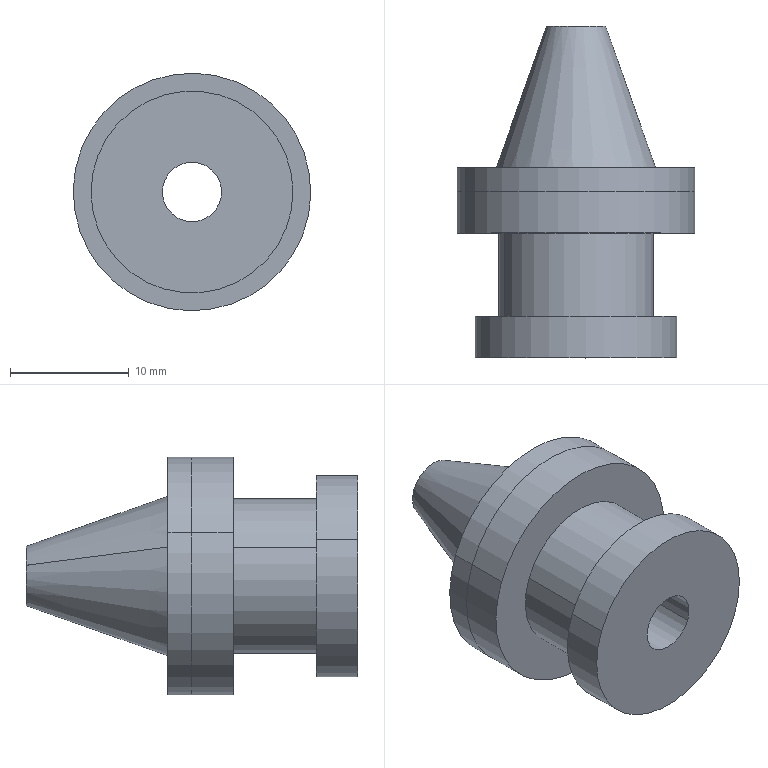Component | SolidWorks | CylinderEndCap-1 | 2 solids | 20 faces | box 20 x 27.94 x 20 mm | volume 3757 mm3 | cylinder 10 | plane 6 | cone 4 | commonest cylinder face diameters 20 x4 5 x2 17 x2 13 x2
build123d program:
from build123d import *

# Parameters (mm, degrees)
SKETCH2_R          = 2.5
CUT_EXTRUDE1_DEPTH = 38.749


with BuildPart() as part:
    # Sketch1 → Revolve1 (revolve)
    with BuildSketch(Plane.XY):
        Polygon((0, 0), (21, 7.436), (21, 10), (24.5, 10), (24.5, 6.5), (31.5, 6.5), (31.5, 8.5), (35, 8.5), (35, 0), align=None)
    revolve(axis=Axis((35, 0, 0), (-1, 0, 0)))

    # Sketch2 → Cut-Extrude1 (cut, through all)
    with BuildSketch(Plane(origin=(35, 0, 0), x_dir=(0, 0, -1), z_dir=(1, 0, 0))):
        with Locations(Location((0, 0, 0), (0, 0, 90))):
            Circle(SKETCH2_R)
    extrude(amount=-CUT_EXTRUDE1_DEPTH, mode=Mode.SUBTRACT)


with BuildPart() as body_2:
    # Sketch3 → Revolve2 (revolve)
    with BuildSketch(Plane.XY):
        Polygon((21, 10), (19, 10), (19, 6.728), (21, 7.436), align=None)
    revolve(axis=Axis((21, 0, 0), (1, 0, 0)))


solid = Compound([part.part, body_2.part])

# Placed as in the assembly
solid = solid.moved(Location((-25, -95, 0), (0, 0, -90)))
STEP:
#1=COLOUR_RGB('',0.7922,0.8196,0.9333);
#2=FILL_AREA_STYLE_COLOUR('',#1);
#3=FILL_AREA_STYLE('',(#2));
#4=SURFACE_STYLE_FILL_AREA(#3);
#5=SURFACE_SIDE_STYLE('',(#4));
#6=SURFACE_STYLE_USAGE(.BOTH.,#5);
#7=PRESENTATION_STYLE_ASSIGNMENT((#6));
#8=CARTESIAN_POINT('',(-0.8926,-4.018,-0.03578));
#9=VERTEX_POINT('',#8);
#10=CARTESIAN_POINT('',(-1.076,-4.018,0.03578));
#11=VERTEX_POINT('',#10);
#12=CARTESIAN_POINT('',(-0.9843,-4.018,0.));
#13=DIRECTION('',(-0.,1.,0.));
#14=DIRECTION('',(0.9316,0.,-0.3635));
#15=AXIS2_PLACEMENT_3D('',#12,#13,#14);
#16=CIRCLE('',#15,0.09843);
#17=EDGE_CURVE('',#9,#11,#16,.T.);
#18=ORIENTED_EDGE('',*,*,#17,.T.);
#19=CARTESIAN_POINT('',(-1.076,-5.118,0.03578));
#20=VERTEX_POINT('',#19);
#21=CARTESIAN_POINT('',(-1.076,-3.74,0.03578));
#22=DIRECTION('',(0.,-1.,0.));
#23=VECTOR('',#22,39.37);
#24=LINE('',#21,#23);
#25=EDGE_CURVE('',#11,#20,#24,.T.);
#26=ORIENTED_EDGE('',*,*,#25,.T.);
#27=CARTESIAN_POINT('',(-0.8926,-5.118,-0.03578));
#28=VERTEX_POINT('',#27);
#29=CARTESIAN_POINT('',(-0.9843,-5.118,0.));
#30=DIRECTION('',(0.,-1.,0.));
#31=DIRECTION('',(0.9316,0.,-0.3635));
#32=AXIS2_PLACEMENT_3D('',#29,#30,#31);
#33=CIRCLE('',#32,0.09843);
#34=EDGE_CURVE('',#20,#28,#33,.T.);
#35=ORIENTED_EDGE('',*,*,#34,.T.);
#36=CARTESIAN_POINT('',(-0.8926,-3.74,-0.03578));
#37=DIRECTION('',(0.,-1.,0.));
#38=VECTOR('',#37,39.37);
#39=LINE('',#36,#38);
#40=EDGE_CURVE('',#9,#28,#39,.T.);
#41=ORIENTED_EDGE('',*,*,#40,.F.);
#42=EDGE_LOOP('',(#18,#26,#35,#41));
#43=FACE_OUTER_BOUND('',#42,.T.);
#44=CARTESIAN_POINT('',(-0.9843,-3.74,0.));
#45=DIRECTION('',(0.,-1.,0.));
#46=DIRECTION('',(0.9316,0.,-0.3635));
#47=AXIS2_PLACEMENT_3D('',#44,#45,#46);
#48=CYLINDRICAL_SURFACE('',#47,0.09843);
#49=ADVANCED_FACE('',(#43),#48,.F.);
#50=CARTESIAN_POINT('',(-0.6725,-4.98,-0.1216));
#51=VERTEX_POINT('',#50);
#52=CARTESIAN_POINT('',(-1.296,-4.98,0.1216));
#53=VERTEX_POINT('',#52);
#54=CARTESIAN_POINT('',(-0.9843,-4.98,0.));
#55=DIRECTION('',(0.,-1.,-0.));
#56=DIRECTION('',(0.9316,0.,-0.3635));
#57=AXIS2_PLACEMENT_3D('',#54,#55,#56);
#58=CIRCLE('',#57,0.3346);
#59=EDGE_CURVE('',#51,#53,#58,.T.);
#60=ORIENTED_EDGE('',*,*,#59,.T.);
#61=CARTESIAN_POINT('',(-1.296,-5.118,0.1216));
#62=VERTEX_POINT('',#61);
#63=CARTESIAN_POINT('',(-1.296,-5.118,0.1216));
#64=DIRECTION('',(0.,-1.,-0.));
#65=VECTOR('',#64,39.37);
#66=LINE('',#63,#65);
#67=EDGE_CURVE('',#53,#62,#66,.T.);
#68=ORIENTED_EDGE('',*,*,#67,.T.);
#69=CARTESIAN_POINT('',(-0.6725,-5.118,-0.1216));
#70=VERTEX_POINT('',#69);
#71=CARTESIAN_POINT('',(-0.9843,-5.118,0.));
#72=DIRECTION('',(0.,-1.,-0.));
#73=DIRECTION('',(0.9316,0.,-0.3635));
#74=AXIS2_PLACEMENT_3D('',#71,#72,#73);
#75=CIRCLE('',#74,0.3346);
#76=EDGE_CURVE('',#70,#62,#75,.T.);
#77=ORIENTED_EDGE('',*,*,#76,.F.);
#78=CARTESIAN_POINT('',(-0.6725,-5.118,-0.1216));
#79=DIRECTION('',(0.,-1.,-0.));
#80=VECTOR('',#79,39.37);
#81=LINE('',#78,#80);
#82=EDGE_CURVE('',#51,#70,#81,.T.);
#83=ORIENTED_EDGE('',*,*,#82,.F.);
#84=EDGE_LOOP('',(#60,#68,#77,#83));
#85=FACE_OUTER_BOUND('',#84,.T.);
#86=CARTESIAN_POINT('',(-0.9843,-5.118,0.));
#87=DIRECTION('',(0.,-1.,-0.));
#88=DIRECTION('',(0.9316,0.,-0.3635));
#89=AXIS2_PLACEMENT_3D('',#86,#87,#88);
#90=CYLINDRICAL_SURFACE('',#89,0.3346);
#91=ADVANCED_FACE('',(#85),#90,.T.);
#92=CARTESIAN_POINT('',(-0.7459,-4.705,-0.09302));
#93=VERTEX_POINT('',#92);
#94=CARTESIAN_POINT('',(-1.223,-4.705,0.09302));
#95=VERTEX_POINT('',#94);
#96=CARTESIAN_POINT('',(-0.9843,-4.705,0.));
#97=DIRECTION('',(0.,-1.,-0.));
#98=DIRECTION('',(0.9316,0.,-0.3635));
#99=AXIS2_PLACEMENT_3D('',#96,#97,#98);
#100=CIRCLE('',#99,0.2559);
#101=EDGE_CURVE('',#93,#95,#100,.T.);
#102=ORIENTED_EDGE('',*,*,#101,.T.);
#103=CARTESIAN_POINT('',(-1.223,-4.98,0.09302));
#104=VERTEX_POINT('',#103);
#105=CARTESIAN_POINT('',(-1.223,-5.118,0.09302));
#106=DIRECTION('',(0.,-1.,-0.));
#107=VECTOR('',#106,39.37);
#108=LINE('',#105,#107);
#109=EDGE_CURVE('',#95,#104,#108,.T.);
#110=ORIENTED_EDGE('',*,*,#109,.T.);
#111=CARTESIAN_POINT('',(-0.7459,-4.98,-0.09302));
#112=VERTEX_POINT('',#111);
#113=CARTESIAN_POINT('',(-0.9843,-4.98,0.));
#114=DIRECTION('',(0.,-1.,-0.));
#115=DIRECTION('',(0.9316,0.,-0.3635));
#116=AXIS2_PLACEMENT_3D('',#113,#114,#115);
#117=CIRCLE('',#116,0.2559);
#118=EDGE_CURVE('',#112,#104,#117,.T.);
#119=ORIENTED_EDGE('',*,*,#118,.F.);
#120=CARTESIAN_POINT('',(-0.7459,-5.118,-0.09302));
#121=DIRECTION('',(0.,-1.,-0.));
#122=VECTOR('',#121,39.37);
#123=LINE('',#120,#122);
#124=EDGE_CURVE('',#93,#112,#123,.T.);
#125=ORIENTED_EDGE('',*,*,#124,.F.);
#126=EDGE_LOOP('',(#102,#110,#119,#125));
#127=FACE_OUTER_BOUND('',#126,.T.);
#128=CARTESIAN_POINT('',(-0.9843,-5.118,0.));
#129=DIRECTION('',(0.,-1.,-0.));
#130=DIRECTION('',(0.9316,0.,-0.3635));
#131=AXIS2_PLACEMENT_3D('',#128,#129,#130);
#132=CYLINDRICAL_SURFACE('',#131,0.2559);
#133=ADVANCED_FACE('',(#127),#132,.T.);
#134=CARTESIAN_POINT('',(-0.6175,-4.567,-0.1431));
#135=VERTEX_POINT('',#134);
#136=CARTESIAN_POINT('',(-1.351,-4.567,0.1431));
#137=VERTEX_POINT('',#136);
#138=CARTESIAN_POINT('',(-0.9843,-4.567,0.));
#139=DIRECTION('',(0.,-1.,-0.));
#140=DIRECTION('',(0.9316,0.,-0.3635));
#141=AXIS2_PLACEMENT_3D('',#138,#139,#140);
#142=CIRCLE('',#141,0.3937);
#143=EDGE_CURVE('',#135,#137,#142,.T.);
#144=ORIENTED_EDGE('',*,*,#143,.T.);
#145=CARTESIAN_POINT('',(-1.351,-4.705,0.1431));
#146=VERTEX_POINT('',#145);
#147=CARTESIAN_POINT('',(-1.351,-5.118,0.1431));
#148=DIRECTION('',(0.,-1.,-0.));
#149=VECTOR('',#148,39.37);
#150=LINE('',#147,#149);
#151=EDGE_CURVE('',#137,#146,#150,.T.);
#152=ORIENTED_EDGE('',*,*,#151,.T.);
#153=CARTESIAN_POINT('',(-0.6175,-4.705,-0.1431));
#154=VERTEX_POINT('',#153);
#155=CARTESIAN_POINT('',(-0.9843,-4.705,0.));
#156=DIRECTION('',(0.,-1.,-0.));
#157=DIRECTION('',(0.9316,0.,-0.3635));
#158=AXIS2_PLACEMENT_3D('',#155,#156,#157);
#159=CIRCLE('',#158,0.3937);
#160=EDGE_CURVE('',#154,#146,#159,.T.);
#161=ORIENTED_EDGE('',*,*,#160,.F.);
#162=CARTESIAN_POINT('',(-0.6175,-5.118,-0.1431));
#163=DIRECTION('',(0.,-1.,-0.));
#164=VECTOR('',#163,39.37);
#165=LINE('',#162,#164);
#166=EDGE_CURVE('',#135,#154,#165,.T.);
#167=ORIENTED_EDGE('',*,*,#166,.F.);
#168=EDGE_LOOP('',(#144,#152,#161,#167));
#169=FACE_OUTER_BOUND('',#168,.T.);
#170=CARTESIAN_POINT('',(-0.9843,-5.118,0.));
#171=DIRECTION('',(0.,-1.,-0.));
#172=DIRECTION('',(0.9316,0.,-0.3635));
#173=AXIS2_PLACEMENT_3D('',#170,#171,#172);
#174=CYLINDRICAL_SURFACE('',#173,0.3937);
#175=ADVANCED_FACE('',(#169),#174,.T.);
#176=CARTESIAN_POINT('',(-0.9843,-4.018,0.));
#177=DIRECTION('',(-0.,1.,0.));
#178=DIRECTION('',(0.9316,0.,-0.3635));
#179=AXIS2_PLACEMENT_3D('',#176,#177,#178);
#180=CIRCLE('',#179,0.09843);
#181=EDGE_CURVE('',#11,#9,#180,.T.);
#182=ORIENTED_EDGE('',*,*,#181,.F.);
#183=CARTESIAN_POINT('',(-1.257,-4.567,0.1064));
#184=VERTEX_POINT('',#183);
#185=CARTESIAN_POINT('',(-1.257,-4.567,0.1064));
#186=DIRECTION('',(-0.311,-0.9426,0.1213));
#187=VECTOR('',#186,39.37);
#188=LINE('',#185,#187);
#189=EDGE_CURVE('',#11,#184,#188,.T.);
#190=ORIENTED_EDGE('',*,*,#189,.T.);
#191=CARTESIAN_POINT('',(-0.7115,-4.567,-0.1064));
#192=VERTEX_POINT('',#191);
#193=CARTESIAN_POINT('',(-0.9843,-4.567,0.));
#194=DIRECTION('',(0.,-1.,-0.));
#195=DIRECTION('',(0.9316,0.,-0.3635));
#196=AXIS2_PLACEMENT_3D('',#193,#194,#195);
#197=CIRCLE('',#196,0.2928);
#198=EDGE_CURVE('',#192,#184,#197,.T.);
#199=ORIENTED_EDGE('',*,*,#198,.F.);
#200=CARTESIAN_POINT('',(-0.7115,-4.567,-0.1064));
#201=DIRECTION('',(0.311,-0.9426,-0.1213));
#202=VECTOR('',#201,39.37);
#203=LINE('',#200,#202);
#204=EDGE_CURVE('',#9,#192,#203,.T.);
#205=ORIENTED_EDGE('',*,*,#204,.F.);
#206=EDGE_LOOP('',(#182,#190,#199,#205));
#207=FACE_OUTER_BOUND('',#206,.T.);
#208=CARTESIAN_POINT('',(-0.9843,-4.567,0.));
#209=DIRECTION('',(0.,-1.,-0.));
#210=DIRECTION('',(0.9316,0.,-0.3635));
#211=AXIS2_PLACEMENT_3D('',#208,#209,#210);
#212=CONICAL_SURFACE('',#211,0.2928,0.3403);
#213=ADVANCED_FACE('',(#207),#212,.T.);
#214=ORIENTED_EDGE('',*,*,#189,.F.);
#215=ORIENTED_EDGE('',*,*,#17,.F.);
#216=ORIENTED_EDGE('',*,*,#204,.T.);
#217=CARTESIAN_POINT('',(-0.9843,-4.567,0.));
#218=DIRECTION('',(0.,-1.,-0.));
#219=DIRECTION('',(0.9316,0.,-0.3635));
#220=AXIS2_PLACEMENT_3D('',#217,#218,#219);
#221=CIRCLE('',#220,0.2928);
#222=EDGE_CURVE('',#184,#192,#221,.T.);
#223=ORIENTED_EDGE('',*,*,#222,.F.);
#224=EDGE_LOOP('',(#214,#215,#216,#223));
#225=FACE_OUTER_BOUND('',#224,.T.);
#226=CARTESIAN_POINT('',(-0.9843,-4.567,0.));
#227=DIRECTION('',(0.,-1.,-0.));
#228=DIRECTION('',(0.9316,0.,-0.3635));
#229=AXIS2_PLACEMENT_3D('',#226,#227,#228);
#230=CONICAL_SURFACE('',#229,0.2928,0.3403);
#231=ADVANCED_FACE('',(#225),#230,.T.);
#232=ORIENTED_EDGE('',*,*,#198,.T.);
#233=ORIENTED_EDGE('',*,*,#222,.T.);
#234=EDGE_LOOP('',(#232,#233));
#235=FACE_BOUND('',#234,.T.);
#236=ORIENTED_EDGE('',*,*,#143,.F.);
#237=CARTESIAN_POINT('',(-0.9843,-4.567,0.));
#238=DIRECTION('',(0.,-1.,-0.));
#239=DIRECTION('',(0.9316,0.,-0.3635));
#240=AXIS2_PLACEMENT_3D('',#237,#238,#239);
#241=CIRCLE('',#240,0.3937);
#242=EDGE_CURVE('',#137,#135,#241,.T.);
#243=ORIENTED_EDGE('',*,*,#242,.F.);
#244=EDGE_LOOP('',(#236,#243));
#245=FACE_OUTER_BOUND('',#244,.T.);
#246=CARTESIAN_POINT('',(-0.7115,-4.567,-0.1064));
#247=DIRECTION('',(-0.,1.,0.));
#248=DIRECTION('',(-0.9316,-0.,0.3635));
#249=AXIS2_PLACEMENT_3D('',#246,#247,#248);
#250=PLANE('',#249);
#251=ADVANCED_FACE('',(#235,#245),#250,.T.);
#252=ORIENTED_EDGE('',*,*,#151,.F.);
#253=ORIENTED_EDGE('',*,*,#242,.T.);
#254=ORIENTED_EDGE('',*,*,#166,.T.);
#255=CARTESIAN_POINT('',(-0.9843,-4.705,0.));
#256=DIRECTION('',(0.,-1.,-0.));
#257=DIRECTION('',(0.9316,0.,-0.3635));
#258=AXIS2_PLACEMENT_3D('',#255,#256,#257);
#259=CIRCLE('',#258,0.3937);
#260=EDGE_CURVE('',#146,#154,#259,.T.);
#261=ORIENTED_EDGE('',*,*,#260,.F.);
#262=EDGE_LOOP('',(#252,#253,#254,#261));
#263=FACE_OUTER_BOUND('',#262,.T.);
#264=CARTESIAN_POINT('',(-0.9843,-5.118,0.));
#265=DIRECTION('',(0.,-1.,-0.));
#266=DIRECTION('',(0.9316,0.,-0.3635));
#267=AXIS2_PLACEMENT_3D('',#264,#265,#266);
#268=CYLINDRICAL_SURFACE('',#267,0.3937);
#269=ADVANCED_FACE('',(#263),#268,.T.);
#270=ORIENTED_EDGE('',*,*,#160,.T.);
#271=ORIENTED_EDGE('',*,*,#260,.T.);
#272=EDGE_LOOP('',(#270,#271));
#273=FACE_OUTER_BOUND('',#272,.T.);
#274=ORIENTED_EDGE('',*,*,#101,.F.);
#275=CARTESIAN_POINT('',(-0.9843,-4.705,0.));
#276=DIRECTION('',(0.,-1.,-0.));
#277=DIRECTION('',(0.9316,0.,-0.3635));
#278=AXIS2_PLACEMENT_3D('',#275,#276,#277);
#279=CIRCLE('',#278,0.2559);
#280=EDGE_CURVE('',#95,#93,#279,.T.);
#281=ORIENTED_EDGE('',*,*,#280,.F.);
#282=EDGE_LOOP('',(#274,#281));
#283=FACE_BOUND('',#282,.T.);
#284=CARTESIAN_POINT('',(-0.6175,-4.705,-0.1431));
#285=DIRECTION('',(0.,-1.,-0.));
#286=DIRECTION('',(0.9316,0.,-0.3635));
#287=AXIS2_PLACEMENT_3D('',#284,#285,#286);
#288=PLANE('',#287);
#289=ADVANCED_FACE('',(#273,#283),#288,.T.);
#290=ORIENTED_EDGE('',*,*,#109,.F.);
#291=ORIENTED_EDGE('',*,*,#280,.T.);
#292=ORIENTED_EDGE('',*,*,#124,.T.);
#293=CARTESIAN_POINT('',(-0.9843,-4.98,0.));
#294=DIRECTION('',(0.,-1.,-0.));
#295=DIRECTION('',(0.9316,0.,-0.3635));
#296=AXIS2_PLACEMENT_3D('',#293,#294,#295);
#297=CIRCLE('',#296,0.2559);
#298=EDGE_CURVE('',#104,#112,#297,.T.);
#299=ORIENTED_EDGE('',*,*,#298,.F.);
#300=EDGE_LOOP('',(#290,#291,#292,#299));
#301=FACE_OUTER_BOUND('',#300,.T.);
#302=CARTESIAN_POINT('',(-0.9843,-5.118,0.));
#303=DIRECTION('',(0.,-1.,-0.));
#304=DIRECTION('',(0.9316,0.,-0.3635));
#305=AXIS2_PLACEMENT_3D('',#302,#303,#304);
#306=CYLINDRICAL_SURFACE('',#305,0.2559);
#307=ADVANCED_FACE('',(#301),#306,.T.);
#308=ORIENTED_EDGE('',*,*,#118,.T.);
#309=ORIENTED_EDGE('',*,*,#298,.T.);
#310=EDGE_LOOP('',(#308,#309));
#311=FACE_BOUND('',#310,.T.);
#312=ORIENTED_EDGE('',*,*,#59,.F.);
#313=CARTESIAN_POINT('',(-0.9843,-4.98,0.));
#314=DIRECTION('',(0.,-1.,-0.));
#315=DIRECTION('',(0.9316,0.,-0.3635));
#316=AXIS2_PLACEMENT_3D('',#313,#314,#315);
#317=CIRCLE('',#316,0.3346);
#318=EDGE_CURVE('',#53,#51,#317,.T.);
#319=ORIENTED_EDGE('',*,*,#318,.F.);
#320=EDGE_LOOP('',(#312,#319));
#321=FACE_OUTER_BOUND('',#320,.T.);
#322=CARTESIAN_POINT('',(-0.7459,-4.98,-0.09302));
#323=DIRECTION('',(-0.,1.,0.));
#324=DIRECTION('',(-0.9316,-0.,0.3635));
#325=AXIS2_PLACEMENT_3D('',#322,#323,#324);
#326=PLANE('',#325);
#327=ADVANCED_FACE('',(#311,#321),#326,.T.);
#328=ORIENTED_EDGE('',*,*,#67,.F.);
#329=ORIENTED_EDGE('',*,*,#318,.T.);
#330=ORIENTED_EDGE('',*,*,#82,.T.);
#331=CARTESIAN_POINT('',(-0.9843,-5.118,0.));
#332=DIRECTION('',(0.,-1.,-0.));
#333=DIRECTION('',(0.9316,0.,-0.3635));
#334=AXIS2_PLACEMENT_3D('',#331,#332,#333);
#335=CIRCLE('',#334,0.3346);
#336=EDGE_CURVE('',#62,#70,#335,.T.);
#337=ORIENTED_EDGE('',*,*,#336,.F.);
#338=EDGE_LOOP('',(#328,#329,#330,#337));
#339=FACE_OUTER_BOUND('',#338,.T.);
#340=CARTESIAN_POINT('',(-0.9843,-5.118,0.));
#341=DIRECTION('',(0.,-1.,-0.));
#342=DIRECTION('',(0.9316,0.,-0.3635));
#343=AXIS2_PLACEMENT_3D('',#340,#341,#342);
#344=CYLINDRICAL_SURFACE('',#343,0.3346);
#345=ADVANCED_FACE('',(#339),#344,.T.);
#346=CARTESIAN_POINT('',(-0.9843,-5.118,0.));
#347=DIRECTION('',(0.,-1.,0.));
#348=DIRECTION('',(0.9316,0.,-0.3635));
#349=AXIS2_PLACEMENT_3D('',#346,#347,#348);
#350=CIRCLE('',#349,0.09843);
#351=EDGE_CURVE('',#28,#20,#350,.T.);
#352=ORIENTED_EDGE('',*,*,#351,.F.);
#353=ORIENTED_EDGE('',*,*,#34,.F.);
#354=EDGE_LOOP('',(#352,#353));
#355=FACE_BOUND('',#354,.T.);
#356=ORIENTED_EDGE('',*,*,#76,.T.);
#357=ORIENTED_EDGE('',*,*,#336,.T.);
#358=EDGE_LOOP('',(#356,#357));
#359=FACE_OUTER_BOUND('',#358,.T.);
#360=CARTESIAN_POINT('',(-0.6725,-5.118,-0.1216));
#361=DIRECTION('',(0.,-1.,-0.));
#362=DIRECTION('',(0.9316,0.,-0.3635));
#363=AXIS2_PLACEMENT_3D('',#360,#361,#362);
#364=PLANE('',#363);
#365=ADVANCED_FACE('',(#355,#359),#364,.T.);
#366=ORIENTED_EDGE('',*,*,#25,.F.);
#367=ORIENTED_EDGE('',*,*,#181,.T.);
#368=ORIENTED_EDGE('',*,*,#40,.T.);
#369=ORIENTED_EDGE('',*,*,#351,.T.);
#370=EDGE_LOOP('',(#366,#367,#368,#369));
#371=FACE_OUTER_BOUND('',#370,.T.);
#372=CARTESIAN_POINT('',(-0.9843,-3.74,0.));
#373=DIRECTION('',(0.,-1.,0.));
#374=DIRECTION('',(0.9316,0.,-0.3635));
#375=AXIS2_PLACEMENT_3D('',#372,#373,#374);
#376=CYLINDRICAL_SURFACE('',#375,0.09843);
#377=ADVANCED_FACE('',(#371),#376,.F.);
#378=CLOSED_SHELL('',(#49,#91,#133,#175,#213,#231,#251,#269,#289,#307,#327,#345,#365,#377));
#379=MANIFOLD_SOLID_BREP('',#378);
#380=STYLED_ITEM('',(#7),#379);
#381=PRESENTATION_LAYER_ASSIGNMENT('','',(#380));
#382=(LENGTH_UNIT()NAMED_UNIT(*)SI_UNIT($,.METRE.));
#383=LENGTH_MEASURE_WITH_UNIT(LENGTH_MEASURE(0.0254),#382);
#384=DIMENSIONAL_EXPONENTS(1.,0.,0.,0.,0.,0.,0.);
#385=(CONVERSION_BASED_UNIT('',#383)LENGTH_UNIT()NAMED_UNIT(#384));
#386=UNCERTAINTY_MEASURE_WITH_UNIT(LENGTH_MEASURE(0.00001),#385,'','');
#387=(NAMED_UNIT(*)PLANE_ANGLE_UNIT()SI_UNIT($,.RADIAN.));
#388=(NAMED_UNIT(*)SI_UNIT($,.STERADIAN.)SOLID_ANGLE_UNIT());
#389=(GEOMETRIC_REPRESENTATION_CONTEXT(3)GLOBAL_UNCERTAINTY_ASSIGNED_CONTEXT((#386))GLOBAL_UNIT_ASSIGNED_CONTEXT((#385,#387,#388))REPRESENTATION_CONTEXT('',''));
#390=MECHANICAL_DESIGN_GEOMETRIC_PRESENTATION_REPRESENTATION('',(#380),#389);
#391=COLOUR_RGB('',0.7922,0.8196,0.9333);
#392=FILL_AREA_STYLE_COLOUR('',#391);
#393=FILL_AREA_STYLE('',(#392));
#394=SURFACE_STYLE_FILL_AREA(#393);
#395=SURFACE_SIDE_STYLE('',(#394));
#396=SURFACE_STYLE_USAGE(.BOTH.,#395);
#397=PRESENTATION_STYLE_ASSIGNMENT((#396));
#398=CARTESIAN_POINT('',(-0.6175,-4.488,-0.1431));
#399=VERTEX_POINT('',#398);
#400=CARTESIAN_POINT('',(-1.351,-4.488,0.1431));
#401=VERTEX_POINT('',#400);
#402=CARTESIAN_POINT('',(-0.9843,-4.488,0.));
#403=DIRECTION('',(0.,-1.,-0.));
#404=DIRECTION('',(0.9316,0.,-0.3635));
#405=AXIS2_PLACEMENT_3D('',#402,#403,#404);
#406=CIRCLE('',#405,0.3937);
#407=EDGE_CURVE('',#399,#401,#406,.T.);
#408=ORIENTED_EDGE('',*,*,#407,.T.);
#409=CARTESIAN_POINT('',(-1.351,-4.567,0.1431));
#410=VERTEX_POINT('',#409);
#411=CARTESIAN_POINT('',(-1.351,-4.567,0.1431));
#412=DIRECTION('',(0.,-1.,-0.));
#413=VECTOR('',#412,39.37);
#414=LINE('',#411,#413);
#415=EDGE_CURVE('',#401,#410,#414,.T.);
#416=ORIENTED_EDGE('',*,*,#415,.T.);
#417=CARTESIAN_POINT('',(-0.6175,-4.567,-0.1431));
#418=VERTEX_POINT('',#417);
#419=CARTESIAN_POINT('',(-0.9843,-4.567,0.));
#420=DIRECTION('',(0.,-1.,-0.));
#421=DIRECTION('',(0.9316,0.,-0.3635));
#422=AXIS2_PLACEMENT_3D('',#419,#420,#421);
#423=CIRCLE('',#422,0.3937);
#424=EDGE_CURVE('',#418,#410,#423,.T.);
#425=ORIENTED_EDGE('',*,*,#424,.F.);
#426=CARTESIAN_POINT('',(-0.6175,-4.567,-0.1431));
#427=DIRECTION('',(0.,-1.,-0.));
#428=VECTOR('',#427,39.37);
#429=LINE('',#426,#428);
#430=EDGE_CURVE('',#399,#418,#429,.T.);
#431=ORIENTED_EDGE('',*,*,#430,.F.);
#432=EDGE_LOOP('',(#408,#416,#425,#431));
#433=FACE_OUTER_BOUND('',#432,.T.);
#434=CARTESIAN_POINT('',(-0.9843,-4.567,0.));
#435=DIRECTION('',(0.,-1.,-0.));
#436=DIRECTION('',(0.9316,0.,-0.3635));
#437=AXIS2_PLACEMENT_3D('',#434,#435,#436);
#438=CYLINDRICAL_SURFACE('',#437,0.3937);
#439=ADVANCED_FACE('',(#433),#438,.T.);
#440=CARTESIAN_POINT('',(-1.231,-4.488,0.09629));
#441=VERTEX_POINT('',#440);
#442=CARTESIAN_POINT('',(-0.7375,-4.488,-0.09629));
#443=VERTEX_POINT('',#442);
#444=CARTESIAN_POINT('',(-0.9843,-4.488,0.));
#445=DIRECTION('',(0.,-1.,-0.));
#446=DIRECTION('',(0.9316,0.,-0.3635));
#447=AXIS2_PLACEMENT_3D('',#444,#445,#446);
#448=CIRCLE('',#447,0.2649);
#449=EDGE_CURVE('',#441,#443,#448,.T.);
#450=ORIENTED_EDGE('',*,*,#449,.F.);
#451=CARTESIAN_POINT('',(-1.257,-4.567,0.1064));
#452=VERTEX_POINT('',#451);
#453=CARTESIAN_POINT('',(-1.231,-4.488,0.09629));
#454=DIRECTION('',(-0.311,-0.9426,0.1213));
#455=VECTOR('',#454,39.37);
#456=LINE('',#453,#455);
#457=EDGE_CURVE('',#441,#452,#456,.T.);
#458=ORIENTED_EDGE('',*,*,#457,.T.);
#459=CARTESIAN_POINT('',(-0.7115,-4.567,-0.1064));
#460=VERTEX_POINT('',#459);
#461=CARTESIAN_POINT('',(-0.9843,-4.567,0.));
#462=DIRECTION('',(0.,-1.,-0.));
#463=DIRECTION('',(0.9316,0.,-0.3635));
#464=AXIS2_PLACEMENT_3D('',#461,#462,#463);
#465=CIRCLE('',#464,0.2928);
#466=EDGE_CURVE('',#452,#460,#465,.T.);
#467=ORIENTED_EDGE('',*,*,#466,.T.);
#468=CARTESIAN_POINT('',(-0.7375,-4.488,-0.09629));
#469=DIRECTION('',(0.311,-0.9426,-0.1213));
#470=VECTOR('',#469,39.37);
#471=LINE('',#468,#470);
#472=EDGE_CURVE('',#443,#460,#471,.T.);
#473=ORIENTED_EDGE('',*,*,#472,.F.);
#474=EDGE_LOOP('',(#450,#458,#467,#473));
#475=FACE_OUTER_BOUND('',#474,.T.);
#476=CARTESIAN_POINT('',(-0.9843,-4.488,0.));
#477=DIRECTION('',(0.,-1.,-0.));
#478=DIRECTION('',(0.9316,0.,-0.3635));
#479=AXIS2_PLACEMENT_3D('',#476,#477,#478);
#480=CONICAL_SURFACE('',#479,0.2649,0.3403);
#481=ADVANCED_FACE('',(#475),#480,.F.);
#482=ORIENTED_EDGE('',*,*,#424,.T.);
#483=CARTESIAN_POINT('',(-0.9843,-4.567,0.));
#484=DIRECTION('',(0.,-1.,-0.));
#485=DIRECTION('',(0.9316,0.,-0.3635));
#486=AXIS2_PLACEMENT_3D('',#483,#484,#485);
#487=CIRCLE('',#486,0.3937);
#488=EDGE_CURVE('',#410,#418,#487,.T.);
#489=ORIENTED_EDGE('',*,*,#488,.T.);
#490=EDGE_LOOP('',(#482,#489));
#491=FACE_OUTER_BOUND('',#490,.T.);
#492=CARTESIAN_POINT('',(-0.9843,-4.567,0.));
#493=DIRECTION('',(0.,-1.,-0.));
#494=DIRECTION('',(0.9316,0.,-0.3635));
#495=AXIS2_PLACEMENT_3D('',#492,#493,#494);
#496=CIRCLE('',#495,0.2928);
#497=EDGE_CURVE('',#460,#452,#496,.T.);
#498=ORIENTED_EDGE('',*,*,#497,.F.);
#499=ORIENTED_EDGE('',*,*,#466,.F.);
#500=EDGE_LOOP('',(#498,#499));
#501=FACE_BOUND('',#500,.T.);
#502=CARTESIAN_POINT('',(-0.6175,-4.567,-0.1431));
#503=DIRECTION('',(0.,-1.,-0.));
#504=DIRECTION('',(0.9316,0.,-0.3635));
#505=AXIS2_PLACEMENT_3D('',#502,#503,#504);
#506=PLANE('',#505);
#507=ADVANCED_FACE('',(#491,#501),#506,.T.);
#508=ORIENTED_EDGE('',*,*,#457,.F.);
#509=CARTESIAN_POINT('',(-0.9843,-4.488,0.));
#510=DIRECTION('',(0.,-1.,-0.));
#511=DIRECTION('',(0.9316,0.,-0.3635));
#512=AXIS2_PLACEMENT_3D('',#509,#510,#511);
#513=CIRCLE('',#512,0.2649);
#514=EDGE_CURVE('',#443,#441,#513,.T.);
#515=ORIENTED_EDGE('',*,*,#514,.F.);
#516=ORIENTED_EDGE('',*,*,#472,.T.);
#517=ORIENTED_EDGE('',*,*,#497,.T.);
#518=EDGE_LOOP('',(#508,#515,#516,#517));
#519=FACE_OUTER_BOUND('',#518,.T.);
#520=CARTESIAN_POINT('',(-0.9843,-4.488,0.));
#521=DIRECTION('',(0.,-1.,-0.));
#522=DIRECTION('',(0.9316,0.,-0.3635));
#523=AXIS2_PLACEMENT_3D('',#520,#521,#522);
#524=CONICAL_SURFACE('',#523,0.2649,0.3403);
#525=ADVANCED_FACE('',(#519),#524,.F.);
#526=ORIENTED_EDGE('',*,*,#514,.T.);
#527=ORIENTED_EDGE('',*,*,#449,.T.);
#528=EDGE_LOOP('',(#526,#527));
#529=FACE_BOUND('',#528,.T.);
#530=ORIENTED_EDGE('',*,*,#407,.F.);
#531=CARTESIAN_POINT('',(-0.9843,-4.488,0.));
#532=DIRECTION('',(0.,-1.,-0.));
#533=DIRECTION('',(0.9316,0.,-0.3635));
#534=AXIS2_PLACEMENT_3D('',#531,#532,#533);
#535=CIRCLE('',#534,0.3937);
#536=EDGE_CURVE('',#401,#399,#535,.T.);
#537=ORIENTED_EDGE('',*,*,#536,.F.);
#538=EDGE_LOOP('',(#530,#537));
#539=FACE_OUTER_BOUND('',#538,.T.);
#540=CARTESIAN_POINT('',(-0.6175,-4.488,-0.1431));
#541=DIRECTION('',(-0.,1.,0.));
#542=DIRECTION('',(-0.9316,-0.,0.3635));
#543=AXIS2_PLACEMENT_3D('',#540,#541,#542);
#544=PLANE('',#543);
#545=ADVANCED_FACE('',(#529,#539),#544,.T.);
#546=ORIENTED_EDGE('',*,*,#415,.F.);
#547=ORIENTED_EDGE('',*,*,#536,.T.);
#548=ORIENTED_EDGE('',*,*,#430,.T.);
#549=ORIENTED_EDGE('',*,*,#488,.F.);
#550=EDGE_LOOP('',(#546,#547,#548,#549));
#551=FACE_OUTER_BOUND('',#550,.T.);
#552=CARTESIAN_POINT('',(-0.9843,-4.567,0.));
#553=DIRECTION('',(0.,-1.,-0.));
#554=DIRECTION('',(0.9316,0.,-0.3635));
#555=AXIS2_PLACEMENT_3D('',#552,#553,#554);
#556=CYLINDRICAL_SURFACE('',#555,0.3937);
#557=ADVANCED_FACE('',(#551),#556,.T.);
#558=CLOSED_SHELL('',(#439,#481,#507,#525,#545,#557));
#559=MANIFOLD_SOLID_BREP('',#558);
#560=STYLED_ITEM('',(#397),#559);
#561=(LENGTH_UNIT()NAMED_UNIT(*)SI_UNIT($,.METRE.));
#562=LENGTH_MEASURE_WITH_UNIT(LENGTH_MEASURE(0.0254),#561);
#563=DIMENSIONAL_EXPONENTS(1.,0.,0.,0.,0.,0.,0.);
#564=(CONVERSION_BASED_UNIT('',#562)LENGTH_UNIT()NAMED_UNIT(#563));
#565=UNCERTAINTY_MEASURE_WITH_UNIT(LENGTH_MEASURE(0.00001),#564,'','');
#566=(NAMED_UNIT(*)PLANE_ANGLE_UNIT()SI_UNIT($,.RADIAN.));
#567=(NAMED_UNIT(*)SI_UNIT($,.STERADIAN.)SOLID_ANGLE_UNIT());
#568=(GEOMETRIC_REPRESENTATION_CONTEXT(3)GLOBAL_UNCERTAINTY_ASSIGNED_CONTEXT((#565))GLOBAL_UNIT_ASSIGNED_CONTEXT((#564,#566,#567))REPRESENTATION_CONTEXT('',''));
#569=MECHANICAL_DESIGN_GEOMETRIC_PRESENTATION_REPRESENTATION('',(#560),#568);
#570=PRESENTATION_LAYER_ASSIGNMENT('','',(#560));
#571=CARTESIAN_POINT('',(0.,0.,0.));
#572=DIRECTION('',(0.,0.,1.));
#573=DIRECTION('',(1.,0.,0.));
#574=AXIS2_PLACEMENT_3D('',#571,#572,#573);
#575=(LENGTH_UNIT()NAMED_UNIT(*)SI_UNIT($,.METRE.));
#576=LENGTH_MEASURE_WITH_UNIT(LENGTH_MEASURE(0.0254),#575);
#577=DIMENSIONAL_EXPONENTS(1.,0.,0.,0.,0.,0.,0.);
#578=(CONVERSION_BASED_UNIT('',#576)LENGTH_UNIT()NAMED_UNIT(#577));
#579=UNCERTAINTY_MEASURE_WITH_UNIT(LENGTH_MEASURE(0.00001),#578,'','');
#580=(NAMED_UNIT(*)PLANE_ANGLE_UNIT()SI_UNIT($,.RADIAN.));
#581=(NAMED_UNIT(*)SI_UNIT($,.STERADIAN.)SOLID_ANGLE_UNIT());
#582=(GEOMETRIC_REPRESENTATION_CONTEXT(3)GLOBAL_UNCERTAINTY_ASSIGNED_CONTEXT((#579))GLOBAL_UNIT_ASSIGNED_CONTEXT((#578,#580,#581))REPRESENTATION_CONTEXT('',''));
#583=ADVANCED_BREP_SHAPE_REPRESENTATION('',(#559,#379,#574),#582);